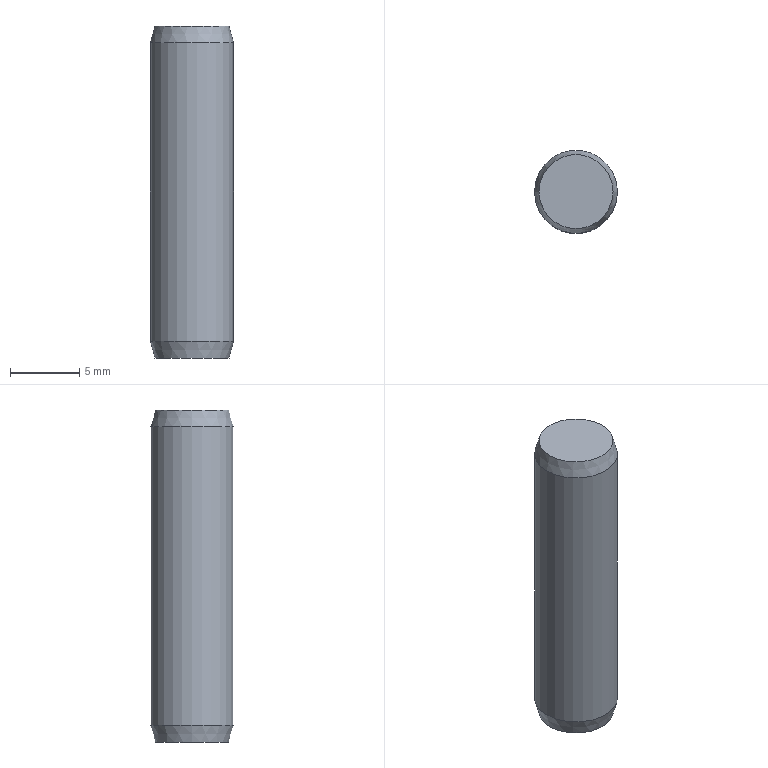Component | NX | GB-T119_1-2000_6X24 | 1 solid | 5 faces | box 6 x 6 x 24 mm | volume 672 mm3 | plane 2 | cone 2 | cylinder 1 | commonest cylinder face diameters 6 x1
STEP:
#1=CARTESIAN_POINT('',(0.,0.,0.));
#2=DIRECTION('',(0.,0.,1.));
#3=DIRECTION('',(1.,0.,0.));
#4=AXIS2_PLACEMENT_3D('',#1,#2,#3);
#5=CARTESIAN_POINT('',(34.322,23.5,-306.5));
#6=VERTEX_POINT('',#5);
#7=CARTESIAN_POINT('',(37.,23.5,-306.5));
#8=DIRECTION('',(0.,0.,-1.));
#9=DIRECTION('',(-1.,0.,0.));
#10=AXIS2_PLACEMENT_3D('',#7,#8,#9);
#11=CIRCLE('',#10,2.678);
#12=CARTESIAN_POINT('',(37.,23.5,-306.5));
#13=DIRECTION('',(0.,0.,-1.));
#14=DIRECTION('',(-1.,0.,0.));
#15=AXIS2_PLACEMENT_3D('',#12,#13,#14);
#16=PLANE('',#15);
#17=CARTESIAN_POINT('',(0.,0.));
#18=DIRECTION('',(1.,0.));
#19=AXIS2_PLACEMENT_2D('',#17,#18);
#20=CIRCLE('',#19,2.678);
#21=(GEOMETRIC_REPRESENTATION_CONTEXT(2)PARAMETRIC_REPRESENTATION_CONTEXT()REPRESENTATION_CONTEXT('',''));
#22=DEFINITIONAL_REPRESENTATION('',(#20),#21);
#23=PCURVE('',#16,#22);
#24=CARTESIAN_POINT('',(37.,23.5,-306.5));
#25=DIRECTION('',(0.,0.,1.));
#26=DIRECTION('',(1.,0.,0.));
#27=AXIS2_PLACEMENT_3D('',#24,#25,#26);
#28=CONICAL_SURFACE('',#27,2.678,0.2618);
#29=CARTESIAN_POINT('',(9.425,-0.));
#30=DIRECTION('',(-1.,0.));
#31=VECTOR('',#30,1.);
#32=LINE('',#29,#31);
#33=(GEOMETRIC_REPRESENTATION_CONTEXT(2)PARAMETRIC_REPRESENTATION_CONTEXT()REPRESENTATION_CONTEXT('',''));
#34=DEFINITIONAL_REPRESENTATION('',(#32),#33);
#35=PCURVE('',#28,#34);
#36=SURFACE_CURVE('',#11,(#23,#35),.PCURVE_S1.);
#37=EDGE_CURVE('',#6,#6,#36,.T.);
#38=ORIENTED_EDGE('',*,*,#37,.T.);
#39=EDGE_LOOP('',(#38));
#40=FACE_BOUND('',#39,.T.);
#41=ADVANCED_FACE('',(#40),#16,.T.);
#42=CARTESIAN_POINT('',(34.,23.5,-305.3));
#43=VERTEX_POINT('',#42);
#44=CARTESIAN_POINT('',(37.,23.5,-305.3));
#45=DIRECTION('',(0.,0.,-1.));
#46=DIRECTION('',(-1.,0.,0.));
#47=AXIS2_PLACEMENT_3D('',#44,#45,#46);
#48=CIRCLE('',#47,3.);
#49=CARTESIAN_POINT('',(9.425,1.2));
#50=DIRECTION('',(-1.,0.));
#51=VECTOR('',#50,1.);
#52=LINE('',#49,#51);
#53=(GEOMETRIC_REPRESENTATION_CONTEXT(2)PARAMETRIC_REPRESENTATION_CONTEXT()REPRESENTATION_CONTEXT('',''));
#54=DEFINITIONAL_REPRESENTATION('',(#52),#53);
#55=PCURVE('',#28,#54);
#56=CARTESIAN_POINT('',(37.,23.5,-282.5));
#57=DIRECTION('',(0.,0.,-1.));
#58=DIRECTION('',(-1.,0.,0.));
#59=AXIS2_PLACEMENT_3D('',#56,#57,#58);
#60=CYLINDRICAL_SURFACE('',#59,3.);
#61=CARTESIAN_POINT('',(0.,22.8));
#62=DIRECTION('',(1.,0.));
#63=VECTOR('',#62,1.);
#64=LINE('',#61,#63);
#65=(GEOMETRIC_REPRESENTATION_CONTEXT(2)PARAMETRIC_REPRESENTATION_CONTEXT()REPRESENTATION_CONTEXT('',''));
#66=DEFINITIONAL_REPRESENTATION('',(#64),#65);
#67=PCURVE('',#60,#66);
#68=SURFACE_CURVE('',#48,(#55,#67),.PCURVE_S1.);
#69=EDGE_CURVE('',#43,#43,#68,.T.);
#70=ORIENTED_EDGE('',*,*,#69,.T.);
#71=CARTESIAN_POINT('',(34.322,23.5,-306.5));
#72=CARTESIAN_POINT('',(34.,23.5,-305.3));
#73=B_SPLINE_CURVE_WITH_KNOTS('',1,(#71,#72),.UNSPECIFIED.,.F.,.F.,(2,2),(-0.,1.242),.PIECEWISE_BEZIER_KNOTS.);
#74=CARTESIAN_POINT('',(3.142,0.));
#75=DIRECTION('',(0.,1.));
#76=VECTOR('',#75,1.);
#77=LINE('',#74,#76);
#78=(GEOMETRIC_REPRESENTATION_CONTEXT(2)PARAMETRIC_REPRESENTATION_CONTEXT()REPRESENTATION_CONTEXT('',''));
#79=DEFINITIONAL_REPRESENTATION('',(#77),#78);
#80=PCURVE('',#28,#79);
#81=CARTESIAN_POINT('',(9.425,0.));
#82=DIRECTION('',(0.,1.));
#83=VECTOR('',#82,1.);
#84=LINE('',#81,#83);
#85=(GEOMETRIC_REPRESENTATION_CONTEXT(2)PARAMETRIC_REPRESENTATION_CONTEXT()REPRESENTATION_CONTEXT('',''));
#86=DEFINITIONAL_REPRESENTATION('',(#84),#85);
#87=PCURVE('',#28,#86);
#88=SEAM_CURVE('',#73,(#80,#87),.PCURVE_S1.);
#89=EDGE_CURVE('',#6,#43,#88,.T.);
#90=ORIENTED_EDGE('',*,*,#89,.F.);
#91=ORIENTED_EDGE('',*,*,#37,.F.);
#92=ORIENTED_EDGE('',*,*,#89,.T.);
#93=EDGE_LOOP('',(#70,#90,#91,#92));
#94=FACE_BOUND('',#93,.T.);
#95=ADVANCED_FACE('',(#94),#28,.T.);
#96=CARTESIAN_POINT('',(34.,23.5,-283.7));
#97=VERTEX_POINT('',#96);
#98=CARTESIAN_POINT('',(37.,23.5,-283.7));
#99=DIRECTION('',(0.,0.,-1.));
#100=DIRECTION('',(-1.,0.,0.));
#101=AXIS2_PLACEMENT_3D('',#98,#99,#100);
#102=CIRCLE('',#101,3.);
#103=CARTESIAN_POINT('',(0.,1.2));
#104=DIRECTION('',(1.,0.));
#105=VECTOR('',#104,1.);
#106=LINE('',#103,#105);
#107=(GEOMETRIC_REPRESENTATION_CONTEXT(2)PARAMETRIC_REPRESENTATION_CONTEXT()REPRESENTATION_CONTEXT('',''));
#108=DEFINITIONAL_REPRESENTATION('',(#106),#107);
#109=PCURVE('',#60,#108);
#110=CARTESIAN_POINT('',(37.,23.5,-283.7));
#111=DIRECTION('',(0.,0.,-1.));
#112=DIRECTION('',(-1.,0.,0.));
#113=AXIS2_PLACEMENT_3D('',#110,#111,#112);
#114=CONICAL_SURFACE('',#113,3.,0.2618);
#115=CARTESIAN_POINT('',(0.,-0.));
#116=DIRECTION('',(1.,0.));
#117=VECTOR('',#116,1.);
#118=LINE('',#115,#117);
#119=(GEOMETRIC_REPRESENTATION_CONTEXT(2)PARAMETRIC_REPRESENTATION_CONTEXT()REPRESENTATION_CONTEXT('',''));
#120=DEFINITIONAL_REPRESENTATION('',(#118),#119);
#121=PCURVE('',#114,#120);
#122=SURFACE_CURVE('',#102,(#109,#121),.PCURVE_S1.);
#123=EDGE_CURVE('',#97,#97,#122,.T.);
#124=ORIENTED_EDGE('',*,*,#123,.T.);
#125=CARTESIAN_POINT('',(34.,23.5,-283.7));
#126=CARTESIAN_POINT('',(34.,23.5,-305.3));
#127=B_SPLINE_CURVE_WITH_KNOTS('',1,(#125,#126),.UNSPECIFIED.,.F.,.F.,(2,2),(1.2,22.8),.PIECEWISE_BEZIER_KNOTS.);
#128=CARTESIAN_POINT('',(6.283,0.));
#129=DIRECTION('',(0.,1.));
#130=VECTOR('',#129,1.);
#131=LINE('',#128,#130);
#132=(GEOMETRIC_REPRESENTATION_CONTEXT(2)PARAMETRIC_REPRESENTATION_CONTEXT()REPRESENTATION_CONTEXT('',''));
#133=DEFINITIONAL_REPRESENTATION('',(#131),#132);
#134=PCURVE('',#60,#133);
#135=CARTESIAN_POINT('',(0.,0.));
#136=DIRECTION('',(0.,1.));
#137=VECTOR('',#136,1.);
#138=LINE('',#135,#137);
#139=(GEOMETRIC_REPRESENTATION_CONTEXT(2)PARAMETRIC_REPRESENTATION_CONTEXT()REPRESENTATION_CONTEXT('',''));
#140=DEFINITIONAL_REPRESENTATION('',(#138),#139);
#141=PCURVE('',#60,#140);
#142=SEAM_CURVE('',#127,(#134,#141),.PCURVE_S1.);
#143=EDGE_CURVE('',#97,#43,#142,.T.);
#144=ORIENTED_EDGE('',*,*,#143,.T.);
#145=ORIENTED_EDGE('',*,*,#69,.F.);
#146=ORIENTED_EDGE('',*,*,#143,.F.);
#147=EDGE_LOOP('',(#124,#144,#145,#146));
#148=FACE_BOUND('',#147,.T.);
#149=ADVANCED_FACE('',(#148),#60,.T.);
#150=CARTESIAN_POINT('',(34.322,23.5,-282.5));
#151=VERTEX_POINT('',#150);
#152=CARTESIAN_POINT('',(37.,23.5,-282.5));
#153=DIRECTION('',(0.,0.,-1.));
#154=DIRECTION('',(-1.,0.,0.));
#155=AXIS2_PLACEMENT_3D('',#152,#153,#154);
#156=CIRCLE('',#155,2.678);
#157=CARTESIAN_POINT('',(0.,-1.2));
#158=DIRECTION('',(1.,0.));
#159=VECTOR('',#158,1.);
#160=LINE('',#157,#159);
#161=(GEOMETRIC_REPRESENTATION_CONTEXT(2)PARAMETRIC_REPRESENTATION_CONTEXT()REPRESENTATION_CONTEXT('',''));
#162=DEFINITIONAL_REPRESENTATION('',(#160),#161);
#163=PCURVE('',#114,#162);
#164=CARTESIAN_POINT('',(39.678,23.5,-282.5));
#165=DIRECTION('',(0.,0.,1.));
#166=DIRECTION('',(1.,0.,0.));
#167=AXIS2_PLACEMENT_3D('',#164,#165,#166);
#168=PLANE('',#167);
#169=CARTESIAN_POINT('',(-5.357,0.));
#170=CARTESIAN_POINT('',(-5.357,4.639));
#171=CARTESIAN_POINT('',(-1.339,2.32));
#172=CARTESIAN_POINT('',(2.678,0.));
#173=CARTESIAN_POINT('',(-1.339,-2.32));
#174=CARTESIAN_POINT('',(-5.357,-4.639));
#175=CARTESIAN_POINT('',(-5.357,0.));
#176=(BOUNDED_CURVE()B_SPLINE_CURVE(2,(#169,#170,#171,#172,#173,#174,#175),.UNSPECIFIED.,.T.,.F.)B_SPLINE_CURVE_WITH_KNOTS((1,2,2,2,2,1),(-2.094,0.,2.094,4.189,6.283,8.378),.UNSPECIFIED.)CURVE()GEOMETRIC_REPRESENTATION_ITEM()RATIONAL_B_SPLINE_CURVE((1.,0.5,1.,0.5,1.,0.5,1.))REPRESENTATION_ITEM(''));
#177=(GEOMETRIC_REPRESENTATION_CONTEXT(2)PARAMETRIC_REPRESENTATION_CONTEXT()REPRESENTATION_CONTEXT('',''));
#178=DEFINITIONAL_REPRESENTATION('',(#176),#177);
#179=PCURVE('',#168,#178);
#180=SURFACE_CURVE('',#156,(#163,#179),.PCURVE_S1.);
#181=EDGE_CURVE('',#151,#151,#180,.T.);
#182=ORIENTED_EDGE('',*,*,#181,.T.);
#183=CARTESIAN_POINT('',(34.322,23.5,-282.5));
#184=CARTESIAN_POINT('',(34.,23.5,-283.7));
#185=B_SPLINE_CURVE_WITH_KNOTS('',1,(#183,#184),.UNSPECIFIED.,.F.,.F.,(2,2),(-1.242,-0.),.PIECEWISE_BEZIER_KNOTS.);
#186=CARTESIAN_POINT('',(6.283,0.));
#187=DIRECTION('',(0.,1.));
#188=VECTOR('',#187,1.);
#189=LINE('',#186,#188);
#190=(GEOMETRIC_REPRESENTATION_CONTEXT(2)PARAMETRIC_REPRESENTATION_CONTEXT()REPRESENTATION_CONTEXT('',''));
#191=DEFINITIONAL_REPRESENTATION('',(#189),#190);
#192=PCURVE('',#114,#191);
#193=CARTESIAN_POINT('',(0.,0.));
#194=DIRECTION('',(0.,1.));
#195=VECTOR('',#194,1.);
#196=LINE('',#193,#195);
#197=(GEOMETRIC_REPRESENTATION_CONTEXT(2)PARAMETRIC_REPRESENTATION_CONTEXT()REPRESENTATION_CONTEXT('',''));
#198=DEFINITIONAL_REPRESENTATION('',(#196),#197);
#199=PCURVE('',#114,#198);
#200=SEAM_CURVE('',#185,(#192,#199),.PCURVE_S1.);
#201=EDGE_CURVE('',#151,#97,#200,.T.);
#202=ORIENTED_EDGE('',*,*,#201,.T.);
#203=ORIENTED_EDGE('',*,*,#123,.F.);
#204=ORIENTED_EDGE('',*,*,#201,.F.);
#205=EDGE_LOOP('',(#182,#202,#203,#204));
#206=FACE_BOUND('',#205,.T.);
#207=ADVANCED_FACE('',(#206),#114,.T.);
#208=ORIENTED_EDGE('',*,*,#181,.F.);
#209=EDGE_LOOP('',(#208));
#210=FACE_BOUND('',#209,.T.);
#211=ADVANCED_FACE('',(#210),#168,.T.);
#212=CLOSED_SHELL('',(#41,#95,#149,#207,#211));
#213=MANIFOLD_SOLID_BREP('',#212);
#214=(LENGTH_UNIT()NAMED_UNIT(*)SI_UNIT(.MILLI.,.METRE.));
#215=UNCERTAINTY_MEASURE_WITH_UNIT(LENGTH_MEASURE(0.00001),#214,'','');
#216=(NAMED_UNIT(*)PLANE_ANGLE_UNIT()SI_UNIT($,.RADIAN.));
#217=(NAMED_UNIT(*)SI_UNIT($,.STERADIAN.)SOLID_ANGLE_UNIT());
#218=(GEOMETRIC_REPRESENTATION_CONTEXT(3)GLOBAL_UNCERTAINTY_ASSIGNED_CONTEXT((#215))GLOBAL_UNIT_ASSIGNED_CONTEXT((#214,#216,#217))REPRESENTATION_CONTEXT('',''));
#219=ADVANCED_BREP_SHAPE_REPRESENTATION('',(#4,#213),#218);